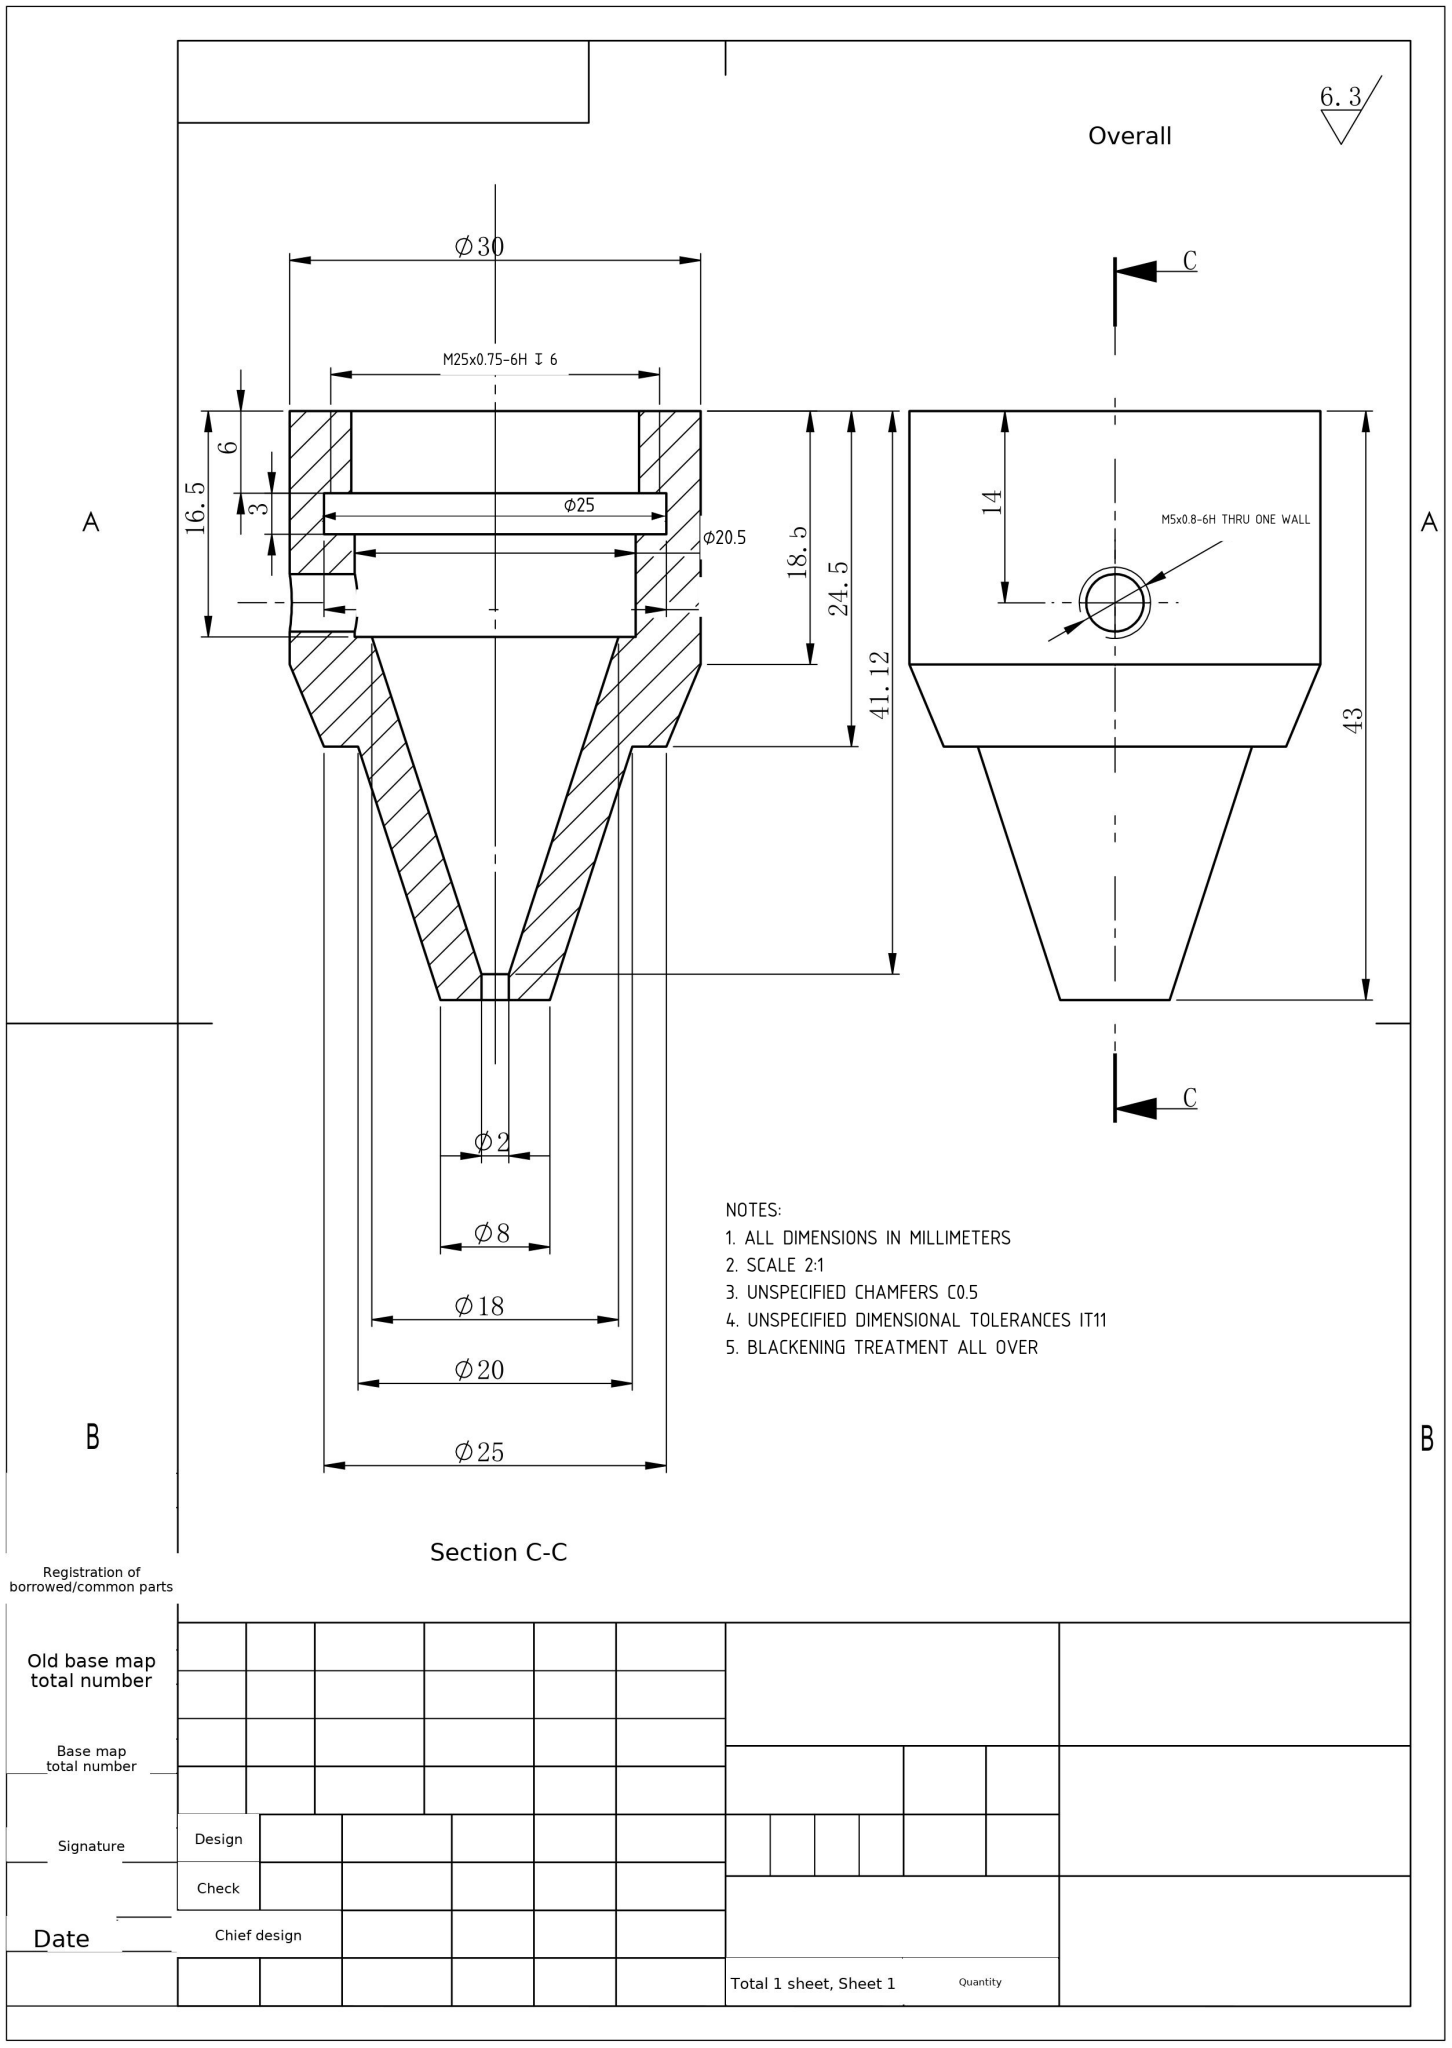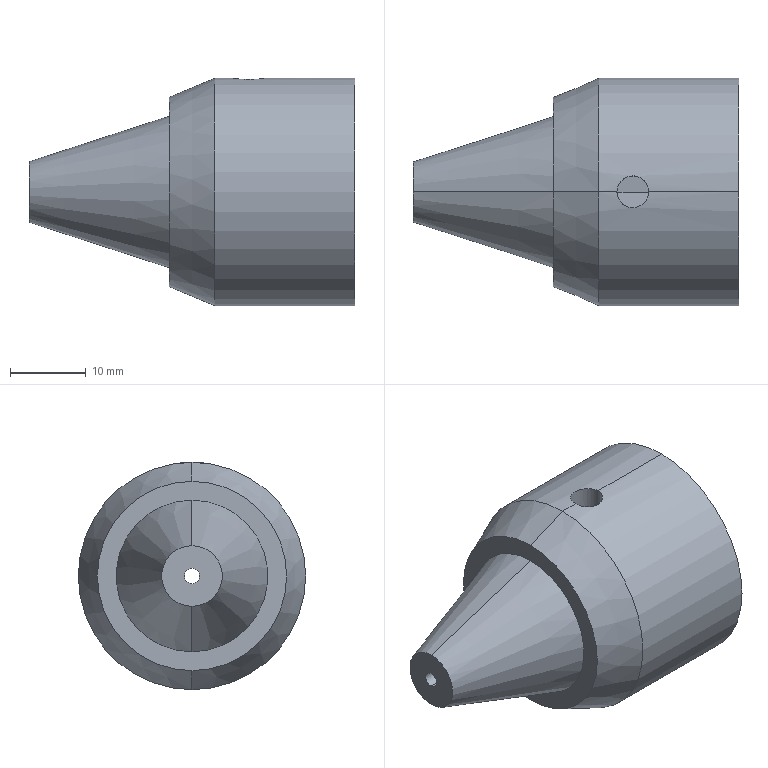Part | NX | mm | 1 solid | 24 faces | box 43 x 30 x 30 mm | volume 11233 mm3 | cylinder 12 | cone 6 | plane 6 | commonest cylinder face diameters 4.2 x2 21 x2 30 x2 2 x2 20.5 x2 25 x2
STEP:
#1=COLOUR_RGB('',0.5294,0.549,0.549);
#2=FILL_AREA_STYLE_COLOUR('',#1);
#3=FILL_AREA_STYLE('',(#2));
#4=SURFACE_STYLE_FILL_AREA(#3);
#5=SURFACE_SIDE_STYLE('',(#4));
#6=SURFACE_STYLE_USAGE(.BOTH.,#5);
#7=PRESENTATION_STYLE_ASSIGNMENT((#6));
#8=CARTESIAN_POINT('',(-9.641,-0.,10.25));
#9=VERTEX_POINT('',#8);
#10=CARTESIAN_POINT('',(-5.441,0.,10.25));
#11=VERTEX_POINT('',#10);
#12=CARTESIAN_POINT('',(-9.641,-0.,10.25));
#13=CARTESIAN_POINT('',(-9.641,-0.2744,10.25));
#14=CARTESIAN_POINT('',(-9.585,-0.5514,10.238));
#15=CARTESIAN_POINT('',(-9.428,-0.9307,10.208));
#16=CARTESIAN_POINT('',(-9.363,-1.053,10.196));
#17=CARTESIAN_POINT('',(-9.21,-1.282,10.17));
#18=CARTESIAN_POINT('',(-9.123,-1.387,10.156));
#19=CARTESIAN_POINT('',(-8.93,-1.581,10.128));
#20=CARTESIAN_POINT('',(-8.822,-1.669,10.113));
#21=CARTESIAN_POINT('',(-8.595,-1.821,10.087));
#22=CARTESIAN_POINT('',(-8.474,-1.886,10.075));
#23=CARTESIAN_POINT('',(-8.092,-2.045,10.045));
#24=CARTESIAN_POINT('',(-7.819,-2.1,10.033));
#25=CARTESIAN_POINT('',(-7.403,-2.1,10.033));
#26=CARTESIAN_POINT('',(-7.267,-2.087,10.035));
#27=CARTESIAN_POINT('',(-6.997,-2.033,10.046));
#28=CARTESIAN_POINT('',(-6.863,-1.993,10.055));
#29=CARTESIAN_POINT('',(-6.61,-1.887,10.075));
#30=CARTESIAN_POINT('',(-6.489,-1.823,10.087));
#31=CARTESIAN_POINT('',(-6.261,-1.67,10.113));
#32=CARTESIAN_POINT('',(-6.153,-1.582,10.128));
#33=CARTESIAN_POINT('',(-5.864,-1.293,10.17));
#34=CARTESIAN_POINT('',(-5.707,-1.059,10.198));
#35=CARTESIAN_POINT('',(-5.549,-0.6807,10.228));
#36=CARTESIAN_POINT('',(-5.509,-0.5474,10.236));
#37=CARTESIAN_POINT('',(-5.454,-0.2764,10.247));
#38=CARTESIAN_POINT('',(-5.441,-0.1391,10.25));
#39=CARTESIAN_POINT('',(-5.441,0.,10.25));
#40=B_SPLINE_CURVE_WITH_KNOTS('',3,(#12,#13,#14,#15,#16,#17,#18,#19,#20,#21,#22,#23,#24,#25,#26,#27,#28,#29,#30,#31,#32,#33,#34,#35,#36,#37,#38,#39),.UNSPECIFIED.,.F.,.F.,(4,2,2,2,2,2,2,2,2,2,2,2,2,4),(0.006583,0.007406,0.007817,0.008228,0.00864,0.009051,0.009874,0.01029,0.0107,0.01111,0.01152,0.01234,0.01275,0.01316),.UNSPECIFIED.);
#41=EDGE_CURVE('',#9,#11,#40,.T.);
#42=ORIENTED_EDGE('',*,*,#41,.F.);
#43=CARTESIAN_POINT('',(-9.641,0.,15.));
#44=VERTEX_POINT('',#43);
#45=CARTESIAN_POINT('',(-9.641,0.,15.));
#46=DIRECTION('',(0.,0.,1.));
#47=VECTOR('',#46,1000.);
#48=LINE('',#45,#47);
#49=EDGE_CURVE('',#9,#44,#48,.T.);
#50=ORIENTED_EDGE('',*,*,#49,.T.);
#51=CARTESIAN_POINT('',(-5.441,0.,15.));
#52=VERTEX_POINT('',#51);
#53=CARTESIAN_POINT('',(-5.441,0.,15.));
#54=CARTESIAN_POINT('',(-5.441,-0.1389,15.));
#55=CARTESIAN_POINT('',(-5.454,-0.2755,14.998));
#56=CARTESIAN_POINT('',(-5.508,-0.5442,14.991));
#57=CARTESIAN_POINT('',(-5.548,-0.6776,14.985));
#58=CARTESIAN_POINT('',(-5.654,-0.9319,14.972));
#59=CARTESIAN_POINT('',(-5.718,-1.052,14.963));
#60=CARTESIAN_POINT('',(-5.871,-1.281,14.946));
#61=CARTESIAN_POINT('',(-5.959,-1.389,14.936));
#62=CARTESIAN_POINT('',(-6.25,-1.679,14.907));
#63=CARTESIAN_POINT('',(-6.484,-1.835,14.888));
#64=CARTESIAN_POINT('',(-6.989,-2.045,14.86));
#65=CARTESIAN_POINT('',(-7.266,-2.1,14.852));
#66=CARTESIAN_POINT('',(-7.677,-2.1,14.852));
#67=CARTESIAN_POINT('',(-7.816,-2.086,14.854));
#68=CARTESIAN_POINT('',(-8.086,-2.033,14.862));
#69=CARTESIAN_POINT('',(-8.217,-1.993,14.867));
#70=CARTESIAN_POINT('',(-8.471,-1.888,14.881));
#71=CARTESIAN_POINT('',(-8.594,-1.822,14.889));
#72=CARTESIAN_POINT('',(-8.821,-1.67,14.907));
#73=CARTESIAN_POINT('',(-8.928,-1.583,14.917));
#74=CARTESIAN_POINT('',(-9.124,-1.387,14.936));
#75=CARTESIAN_POINT('',(-9.21,-1.281,14.946));
#76=CARTESIAN_POINT('',(-9.362,-1.054,14.963));
#77=CARTESIAN_POINT('',(-9.428,-0.9311,14.972));
#78=CARTESIAN_POINT('',(-9.533,-0.6769,14.985));
#79=CARTESIAN_POINT('',(-9.573,-0.5459,14.991));
#80=CARTESIAN_POINT('',(-9.627,-0.2765,14.998));
#81=CARTESIAN_POINT('',(-9.641,-0.1371,15.));
#82=CARTESIAN_POINT('',(-9.641,0.,15.));
#83=B_SPLINE_CURVE_WITH_KNOTS('',3,(#53,#54,#55,#56,#57,#58,#59,#60,#61,#62,#63,#64,#65,#66,#67,#68,#69,#70,#71,#72,#73,#74,#75,#76,#77,#78,#79,#80,#81,#82),.UNSPECIFIED.,.F.,.F.,(4,2,2,2,2,2,2,2,2,2,2,2,2,2,4),(0.,0.0004109,0.0008217,0.001233,0.001643,0.002465,0.003287,0.003698,0.004109,0.004519,0.00493,0.005341,0.005752,0.006163,0.006574),.UNSPECIFIED.);
#84=EDGE_CURVE('',#52,#44,#83,.T.);
#85=ORIENTED_EDGE('',*,*,#84,.F.);
#86=CARTESIAN_POINT('',(-5.441,0.,15.));
#87=DIRECTION('',(0.,0.,1.));
#88=VECTOR('',#87,1000.);
#89=LINE('',#86,#88);
#90=EDGE_CURVE('',#11,#52,#89,.T.);
#91=ORIENTED_EDGE('',*,*,#90,.F.);
#92=EDGE_LOOP('',(#42,#50,#85,#91));
#93=FACE_OUTER_BOUND('',#92,.T.);
#94=CARTESIAN_POINT('',(-7.541,0.,15.));
#95=DIRECTION('',(0.,0.,1.));
#96=DIRECTION('',(1.,0.,0.));
#97=AXIS2_PLACEMENT_3D('',#94,#95,#96);
#98=CYLINDRICAL_SURFACE('',#97,2.1);
#99=ADVANCED_FACE('',(#93),#98,.F.);
#100=CARTESIAN_POINT('',(0.4592,0.,10.5));
#101=VERTEX_POINT('',#100);
#102=CARTESIAN_POINT('',(0.4592,0.,-10.5));
#103=VERTEX_POINT('',#102);
#104=CARTESIAN_POINT('',(0.4592,0.,0.));
#105=DIRECTION('',(1.,0.,0.));
#106=DIRECTION('',(0.,0.,-1.));
#107=AXIS2_PLACEMENT_3D('',#104,#105,#106);
#108=CIRCLE('',#107,10.5);
#109=EDGE_CURVE('',#101,#103,#108,.T.);
#110=ORIENTED_EDGE('',*,*,#109,.F.);
#111=CARTESIAN_POINT('',(6.459,0.,10.5));
#112=VERTEX_POINT('',#111);
#113=CARTESIAN_POINT('',(6.459,0.,10.5));
#114=DIRECTION('',(1.,0.,0.));
#115=VECTOR('',#114,1000.);
#116=LINE('',#113,#115);
#117=EDGE_CURVE('',#101,#112,#116,.T.);
#118=ORIENTED_EDGE('',*,*,#117,.T.);
#119=CARTESIAN_POINT('',(6.459,0.,-10.5));
#120=VERTEX_POINT('',#119);
#121=CARTESIAN_POINT('',(6.459,0.,0.));
#122=DIRECTION('',(1.,0.,0.));
#123=DIRECTION('',(0.,0.,-1.));
#124=AXIS2_PLACEMENT_3D('',#121,#122,#123);
#125=CIRCLE('',#124,10.5);
#126=EDGE_CURVE('',#112,#120,#125,.T.);
#127=ORIENTED_EDGE('',*,*,#126,.T.);
#128=CARTESIAN_POINT('',(6.459,0.,-10.5));
#129=DIRECTION('',(1.,0.,0.));
#130=VECTOR('',#129,1000.);
#131=LINE('',#128,#130);
#132=EDGE_CURVE('',#103,#120,#131,.T.);
#133=ORIENTED_EDGE('',*,*,#132,.F.);
#134=EDGE_LOOP('',(#110,#118,#127,#133));
#135=FACE_OUTER_BOUND('',#134,.T.);
#136=CARTESIAN_POINT('',(6.459,0.,0.));
#137=DIRECTION('',(1.,0.,0.));
#138=DIRECTION('',(0.,0.,-1.));
#139=AXIS2_PLACEMENT_3D('',#136,#137,#138);
#140=CYLINDRICAL_SURFACE('',#139,10.5);
#141=ADVANCED_FACE('',(#135),#140,.F.);
#142=CARTESIAN_POINT('',(6.459,0.,15.));
#143=VERTEX_POINT('',#142);
#144=CARTESIAN_POINT('',(6.459,0.,-15.));
#145=VERTEX_POINT('',#144);
#146=CARTESIAN_POINT('',(6.459,0.,0.));
#147=DIRECTION('',(-1.,0.,0.));
#148=DIRECTION('',(0.,0.,1.));
#149=AXIS2_PLACEMENT_3D('',#146,#147,#148);
#150=CIRCLE('',#149,15.);
#151=EDGE_CURVE('',#143,#145,#150,.T.);
#152=ORIENTED_EDGE('',*,*,#151,.T.);
#153=CARTESIAN_POINT('',(-12.041,0.,-15.));
#154=VERTEX_POINT('',#153);
#155=CARTESIAN_POINT('',(-39.391,0.,-15.));
#156=DIRECTION('',(-1.,0.,0.));
#157=VECTOR('',#156,1000.);
#158=LINE('',#155,#157);
#159=EDGE_CURVE('',#145,#154,#158,.T.);
#160=ORIENTED_EDGE('',*,*,#159,.T.);
#161=CARTESIAN_POINT('',(-12.041,0.,15.));
#162=VERTEX_POINT('',#161);
#163=CARTESIAN_POINT('',(-12.041,0.,0.));
#164=DIRECTION('',(-1.,0.,0.));
#165=DIRECTION('',(0.,0.,1.));
#166=AXIS2_PLACEMENT_3D('',#163,#164,#165);
#167=CIRCLE('',#166,15.);
#168=EDGE_CURVE('',#162,#154,#167,.T.);
#169=ORIENTED_EDGE('',*,*,#168,.F.);
#170=CARTESIAN_POINT('',(-39.391,0.,15.));
#171=DIRECTION('',(-1.,0.,0.));
#172=VECTOR('',#171,1000.);
#173=LINE('',#170,#172);
#174=EDGE_CURVE('',#44,#162,#173,.T.);
#175=ORIENTED_EDGE('',*,*,#174,.F.);
#176=CARTESIAN_POINT('',(-9.641,0.,15.));
#177=CARTESIAN_POINT('',(-9.641,0.2742,15.));
#178=CARTESIAN_POINT('',(-9.586,0.5508,14.992));
#179=CARTESIAN_POINT('',(-9.429,0.9299,14.972));
#180=CARTESIAN_POINT('',(-9.363,1.052,14.963));
#181=CARTESIAN_POINT('',(-9.21,1.281,14.946));
#182=CARTESIAN_POINT('',(-9.123,1.387,14.936));
#183=CARTESIAN_POINT('',(-8.93,1.581,14.917));
#184=CARTESIAN_POINT('',(-8.822,1.669,14.907));
#185=CARTESIAN_POINT('',(-8.594,1.822,14.889));
#186=CARTESIAN_POINT('',(-8.474,1.886,14.881));
#187=CARTESIAN_POINT('',(-8.219,1.992,14.867));
#188=CARTESIAN_POINT('',(-8.086,2.033,14.862));
#189=CARTESIAN_POINT('',(-7.818,2.086,14.854));
#190=CARTESIAN_POINT('',(-7.681,2.1,14.852));
#191=CARTESIAN_POINT('',(-7.403,2.1,14.852));
#192=CARTESIAN_POINT('',(-7.267,2.087,14.854));
#193=CARTESIAN_POINT('',(-6.998,2.033,14.862));
#194=CARTESIAN_POINT('',(-6.865,1.993,14.867));
#195=CARTESIAN_POINT('',(-6.61,1.888,14.881));
#196=CARTESIAN_POINT('',(-6.49,1.823,14.889));
#197=CARTESIAN_POINT('',(-6.262,1.671,14.907));
#198=CARTESIAN_POINT('',(-6.154,1.583,14.917));
#199=CARTESIAN_POINT('',(-5.863,1.293,14.945));
#200=CARTESIAN_POINT('',(-5.707,1.059,14.965));
#201=CARTESIAN_POINT('',(-5.497,0.5538,14.992));
#202=CARTESIAN_POINT('',(-5.441,0.2778,15.));
#203=CARTESIAN_POINT('',(-5.441,0.,15.));
#204=B_SPLINE_CURVE_WITH_KNOTS('',3,(#176,#177,#178,#179,#180,#181,#182,#183,#184,#185,#186,#187,#188,#189,#190,#191,#192,#193,#194,#195,#196,#197,#198,#199,#200,#201,#202,#203),.UNSPECIFIED.,.F.,.F.,(4,2,2,2,2,2,2,2,2,2,2,2,2,4),(0.006574,0.007395,0.007806,0.008217,0.008627,0.009038,0.009449,0.00986,0.01027,0.01068,0.01109,0.0115,0.01232,0.01315),.UNSPECIFIED.);
#205=EDGE_CURVE('',#44,#52,#204,.T.);
#206=ORIENTED_EDGE('',*,*,#205,.T.);
#207=CARTESIAN_POINT('',(-39.391,0.,15.));
#208=DIRECTION('',(-1.,0.,0.));
#209=VECTOR('',#208,1000.);
#210=LINE('',#207,#209);
#211=EDGE_CURVE('',#143,#52,#210,.T.);
#212=ORIENTED_EDGE('',*,*,#211,.F.);
#213=EDGE_LOOP('',(#152,#160,#169,#175,#206,#212));
#214=FACE_OUTER_BOUND('',#213,.T.);
#215=CARTESIAN_POINT('',(-39.391,0.,0.));
#216=DIRECTION('',(-1.,0.,0.));
#217=DIRECTION('',(0.,0.,1.));
#218=AXIS2_PLACEMENT_3D('',#215,#216,#217);
#219=CYLINDRICAL_SURFACE('',#218,15.);
#220=ADVANCED_FACE('',(#214),#219,.T.);
#221=CARTESIAN_POINT('',(-18.041,0.,12.5));
#222=VERTEX_POINT('',#221);
#223=CARTESIAN_POINT('',(-18.041,0.,-12.5));
#224=VERTEX_POINT('',#223);
#225=CARTESIAN_POINT('',(-18.041,0.,0.));
#226=DIRECTION('',(-1.,0.,0.));
#227=DIRECTION('',(0.,0.,1.));
#228=AXIS2_PLACEMENT_3D('',#225,#226,#227);
#229=CIRCLE('',#228,12.5);
#230=EDGE_CURVE('',#222,#224,#229,.T.);
#231=ORIENTED_EDGE('',*,*,#230,.F.);
#232=CARTESIAN_POINT('',(-12.041,0.,15.));
#233=DIRECTION('',(0.9231,0.,0.3846));
#234=VECTOR('',#233,1000.);
#235=LINE('',#232,#234);
#236=EDGE_CURVE('',#222,#162,#235,.T.);
#237=ORIENTED_EDGE('',*,*,#236,.T.);
#238=ORIENTED_EDGE('',*,*,#168,.T.);
#239=CARTESIAN_POINT('',(-12.041,0.,-15.));
#240=DIRECTION('',(0.9231,0.,-0.3846));
#241=VECTOR('',#240,1000.);
#242=LINE('',#239,#241);
#243=EDGE_CURVE('',#224,#154,#242,.T.);
#244=ORIENTED_EDGE('',*,*,#243,.F.);
#245=EDGE_LOOP('',(#231,#237,#238,#244));
#246=FACE_OUTER_BOUND('',#245,.T.);
#247=CARTESIAN_POINT('',(-12.041,0.,0.));
#248=DIRECTION('',(1.,0.,0.));
#249=DIRECTION('',(0.,0.,-1.));
#250=AXIS2_PLACEMENT_3D('',#247,#248,#249);
#251=CONICAL_SURFACE('',#250,15.,0.3948);
#252=ADVANCED_FACE('',(#246),#251,.T.);
#253=CARTESIAN_POINT('',(-36.541,0.,4.));
#254=VERTEX_POINT('',#253);
#255=CARTESIAN_POINT('',(-36.541,0.,-4.));
#256=VERTEX_POINT('',#255);
#257=CARTESIAN_POINT('',(-36.541,0.,0.));
#258=DIRECTION('',(-1.,0.,0.));
#259=DIRECTION('',(0.,0.,1.));
#260=AXIS2_PLACEMENT_3D('',#257,#258,#259);
#261=CIRCLE('',#260,4.);
#262=EDGE_CURVE('',#254,#256,#261,.T.);
#263=ORIENTED_EDGE('',*,*,#262,.F.);
#264=CARTESIAN_POINT('',(-18.041,0.,10.011));
#265=VERTEX_POINT('',#264);
#266=CARTESIAN_POINT('',(-18.041,0.,10.011));
#267=DIRECTION('',(0.9511,0.,0.309));
#268=VECTOR('',#267,1000.);
#269=LINE('',#266,#268);
#270=EDGE_CURVE('',#254,#265,#269,.T.);
#271=ORIENTED_EDGE('',*,*,#270,.T.);
#272=CARTESIAN_POINT('',(-18.041,0.,-10.011));
#273=VERTEX_POINT('',#272);
#274=CARTESIAN_POINT('',(-18.041,0.,0.));
#275=DIRECTION('',(-1.,0.,0.));
#276=DIRECTION('',(0.,0.,1.));
#277=AXIS2_PLACEMENT_3D('',#274,#275,#276);
#278=CIRCLE('',#277,10.011);
#279=EDGE_CURVE('',#265,#273,#278,.T.);
#280=ORIENTED_EDGE('',*,*,#279,.T.);
#281=CARTESIAN_POINT('',(-18.041,0.,-10.011));
#282=DIRECTION('',(0.9511,0.,-0.309));
#283=VECTOR('',#282,1000.);
#284=LINE('',#281,#283);
#285=EDGE_CURVE('',#256,#273,#284,.T.);
#286=ORIENTED_EDGE('',*,*,#285,.F.);
#287=EDGE_LOOP('',(#263,#271,#280,#286));
#288=FACE_OUTER_BOUND('',#287,.T.);
#289=CARTESIAN_POINT('',(-18.041,0.,0.));
#290=DIRECTION('',(1.,0.,0.));
#291=DIRECTION('',(0.,0.,-1.));
#292=AXIS2_PLACEMENT_3D('',#289,#290,#291);
#293=CONICAL_SURFACE('',#292,10.011,0.3142);
#294=ADVANCED_FACE('',(#288),#293,.T.);
#295=CARTESIAN_POINT('',(-34.662,0.,-1.));
#296=VERTEX_POINT('',#295);
#297=CARTESIAN_POINT('',(-34.662,0.,1.));
#298=VERTEX_POINT('',#297);
#299=CARTESIAN_POINT('',(-34.662,0.,0.));
#300=DIRECTION('',(-1.,0.,0.));
#301=DIRECTION('',(0.,0.,1.));
#302=AXIS2_PLACEMENT_3D('',#299,#300,#301);
#303=CIRCLE('',#302,1.);
#304=EDGE_CURVE('',#296,#298,#303,.T.);
#305=ORIENTED_EDGE('',*,*,#304,.F.);
#306=CARTESIAN_POINT('',(-36.541,0.,-1.));
#307=VERTEX_POINT('',#306);
#308=CARTESIAN_POINT('',(-39.391,0.,-1.));
#309=DIRECTION('',(-1.,0.,0.));
#310=VECTOR('',#309,1000.);
#311=LINE('',#308,#310);
#312=EDGE_CURVE('',#296,#307,#311,.T.);
#313=ORIENTED_EDGE('',*,*,#312,.T.);
#314=CARTESIAN_POINT('',(-36.541,0.,1.));
#315=VERTEX_POINT('',#314);
#316=CARTESIAN_POINT('',(-36.541,0.,0.));
#317=DIRECTION('',(-1.,0.,0.));
#318=DIRECTION('',(0.,0.,1.));
#319=AXIS2_PLACEMENT_3D('',#316,#317,#318);
#320=CIRCLE('',#319,1.);
#321=EDGE_CURVE('',#307,#315,#320,.T.);
#322=ORIENTED_EDGE('',*,*,#321,.T.);
#323=CARTESIAN_POINT('',(-39.391,0.,1.));
#324=DIRECTION('',(-1.,0.,0.));
#325=VECTOR('',#324,1000.);
#326=LINE('',#323,#325);
#327=EDGE_CURVE('',#298,#315,#326,.T.);
#328=ORIENTED_EDGE('',*,*,#327,.F.);
#329=EDGE_LOOP('',(#305,#313,#322,#328));
#330=FACE_OUTER_BOUND('',#329,.T.);
#331=CARTESIAN_POINT('',(-39.391,0.,0.));
#332=DIRECTION('',(-1.,0.,0.));
#333=DIRECTION('',(0.,0.,1.));
#334=AXIS2_PLACEMENT_3D('',#331,#332,#333);
#335=CYLINDRICAL_SURFACE('',#334,1.);
#336=ADVANCED_FACE('',(#330),#335,.F.);
#337=ORIENTED_EDGE('',*,*,#304,.T.);
#338=CARTESIAN_POINT('',(-10.041,0.,9.));
#339=VERTEX_POINT('',#338);
#340=CARTESIAN_POINT('',(-34.662,0.,1.));
#341=DIRECTION('',(0.9511,0.,0.309));
#342=VECTOR('',#341,1000.);
#343=LINE('',#340,#342);
#344=EDGE_CURVE('',#298,#339,#343,.T.);
#345=ORIENTED_EDGE('',*,*,#344,.T.);
#346=CARTESIAN_POINT('',(-10.041,0.,-9.));
#347=VERTEX_POINT('',#346);
#348=CARTESIAN_POINT('',(-10.041,0.,0.));
#349=DIRECTION('',(-1.,0.,0.));
#350=DIRECTION('',(0.,0.,1.));
#351=AXIS2_PLACEMENT_3D('',#348,#349,#350);
#352=CIRCLE('',#351,9.);
#353=EDGE_CURVE('',#347,#339,#352,.T.);
#354=ORIENTED_EDGE('',*,*,#353,.F.);
#355=CARTESIAN_POINT('',(-34.662,0.,-1.));
#356=DIRECTION('',(0.9511,0.,-0.309));
#357=VECTOR('',#356,1000.);
#358=LINE('',#355,#357);
#359=EDGE_CURVE('',#296,#347,#358,.T.);
#360=ORIENTED_EDGE('',*,*,#359,.F.);
#361=EDGE_LOOP('',(#337,#345,#354,#360));
#362=FACE_OUTER_BOUND('',#361,.T.);
#363=CARTESIAN_POINT('',(-34.662,0.,0.));
#364=DIRECTION('',(1.,0.,0.));
#365=DIRECTION('',(0.,0.,-1.));
#366=AXIS2_PLACEMENT_3D('',#363,#364,#365);
#367=CONICAL_SURFACE('',#366,1.,0.3142);
#368=ADVANCED_FACE('',(#362),#367,.F.);
#369=CARTESIAN_POINT('',(-2.541,0.,-10.25));
#370=VERTEX_POINT('',#369);
#371=CARTESIAN_POINT('',(-2.541,0.,10.25));
#372=VERTEX_POINT('',#371);
#373=CARTESIAN_POINT('',(-2.541,0.,0.));
#374=DIRECTION('',(-1.,0.,0.));
#375=DIRECTION('',(0.,0.,1.));
#376=AXIS2_PLACEMENT_3D('',#373,#374,#375);
#377=CIRCLE('',#376,10.25);
#378=EDGE_CURVE('',#370,#372,#377,.T.);
#379=ORIENTED_EDGE('',*,*,#378,.F.);
#380=CARTESIAN_POINT('',(-10.041,0.,-10.25));
#381=VERTEX_POINT('',#380);
#382=CARTESIAN_POINT('',(-39.391,0.,-10.25));
#383=DIRECTION('',(-1.,0.,0.));
#384=VECTOR('',#383,1000.);
#385=LINE('',#382,#384);
#386=EDGE_CURVE('',#370,#381,#385,.T.);
#387=ORIENTED_EDGE('',*,*,#386,.T.);
#388=CARTESIAN_POINT('',(-10.041,0.,10.25));
#389=VERTEX_POINT('',#388);
#390=CARTESIAN_POINT('',(-10.041,0.,0.));
#391=DIRECTION('',(-1.,0.,0.));
#392=DIRECTION('',(0.,0.,1.));
#393=AXIS2_PLACEMENT_3D('',#390,#391,#392);
#394=CIRCLE('',#393,10.25);
#395=EDGE_CURVE('',#381,#389,#394,.T.);
#396=ORIENTED_EDGE('',*,*,#395,.T.);
#397=CARTESIAN_POINT('',(-39.391,0.,10.25));
#398=DIRECTION('',(-1.,0.,0.));
#399=VECTOR('',#398,1000.);
#400=LINE('',#397,#399);
#401=EDGE_CURVE('',#9,#389,#400,.T.);
#402=ORIENTED_EDGE('',*,*,#401,.F.);
#403=ORIENTED_EDGE('',*,*,#41,.T.);
#404=CARTESIAN_POINT('',(-39.391,0.,10.25));
#405=DIRECTION('',(-1.,0.,0.));
#406=VECTOR('',#405,1000.);
#407=LINE('',#404,#406);
#408=EDGE_CURVE('',#372,#11,#407,.T.);
#409=ORIENTED_EDGE('',*,*,#408,.F.);
#410=EDGE_LOOP('',(#379,#387,#396,#402,#403,#409));
#411=FACE_OUTER_BOUND('',#410,.T.);
#412=CARTESIAN_POINT('',(-39.391,0.,0.));
#413=DIRECTION('',(-1.,0.,0.));
#414=DIRECTION('',(0.,0.,1.));
#415=AXIS2_PLACEMENT_3D('',#412,#413,#414);
#416=CYLINDRICAL_SURFACE('',#415,10.25);
#417=ADVANCED_FACE('',(#411),#416,.F.);
#418=CARTESIAN_POINT('',(0.4592,0.,-12.5));
#419=VERTEX_POINT('',#418);
#420=CARTESIAN_POINT('',(0.4592,0.,12.5));
#421=VERTEX_POINT('',#420);
#422=CARTESIAN_POINT('',(0.4592,0.,0.));
#423=DIRECTION('',(-1.,0.,0.));
#424=DIRECTION('',(0.,0.,1.));
#425=AXIS2_PLACEMENT_3D('',#422,#423,#424);
#426=CIRCLE('',#425,12.5);
#427=EDGE_CURVE('',#419,#421,#426,.T.);
#428=ORIENTED_EDGE('',*,*,#427,.F.);
#429=CARTESIAN_POINT('',(-2.541,0.,-12.5));
#430=VERTEX_POINT('',#429);
#431=CARTESIAN_POINT('',(-39.391,0.,-12.5));
#432=DIRECTION('',(-1.,0.,0.));
#433=VECTOR('',#432,1000.);
#434=LINE('',#431,#433);
#435=EDGE_CURVE('',#419,#430,#434,.T.);
#436=ORIENTED_EDGE('',*,*,#435,.T.);
#437=CARTESIAN_POINT('',(-2.541,0.,12.5));
#438=VERTEX_POINT('',#437);
#439=CARTESIAN_POINT('',(-2.541,0.,0.));
#440=DIRECTION('',(-1.,0.,0.));
#441=DIRECTION('',(0.,0.,1.));
#442=AXIS2_PLACEMENT_3D('',#439,#440,#441);
#443=CIRCLE('',#442,12.5);
#444=EDGE_CURVE('',#430,#438,#443,.T.);
#445=ORIENTED_EDGE('',*,*,#444,.T.);
#446=CARTESIAN_POINT('',(-39.391,0.,12.5));
#447=DIRECTION('',(-1.,0.,0.));
#448=VECTOR('',#447,1000.);
#449=LINE('',#446,#448);
#450=EDGE_CURVE('',#421,#438,#449,.T.);
#451=ORIENTED_EDGE('',*,*,#450,.F.);
#452=EDGE_LOOP('',(#428,#436,#445,#451));
#453=FACE_OUTER_BOUND('',#452,.T.);
#454=CARTESIAN_POINT('',(-39.391,0.,0.));
#455=DIRECTION('',(-1.,0.,0.));
#456=DIRECTION('',(0.,0.,1.));
#457=AXIS2_PLACEMENT_3D('',#454,#455,#456);
#458=CYLINDRICAL_SURFACE('',#457,12.5);
#459=ADVANCED_FACE('',(#453),#458,.F.);
#460=CARTESIAN_POINT('',(6.459,0.,0.));
#461=DIRECTION('',(1.,0.,0.));
#462=DIRECTION('',(0.,0.,-1.));
#463=AXIS2_PLACEMENT_3D('',#460,#461,#462);
#464=CIRCLE('',#463,10.5);
#465=EDGE_CURVE('',#120,#112,#464,.T.);
#466=ORIENTED_EDGE('',*,*,#465,.F.);
#467=ORIENTED_EDGE('',*,*,#126,.F.);
#468=EDGE_LOOP('',(#466,#467));
#469=FACE_BOUND('',#468,.T.);
#470=ORIENTED_EDGE('',*,*,#151,.F.);
#471=CARTESIAN_POINT('',(6.459,0.,0.));
#472=DIRECTION('',(-1.,0.,0.));
#473=DIRECTION('',(0.,0.,1.));
#474=AXIS2_PLACEMENT_3D('',#471,#472,#473);
#475=CIRCLE('',#474,15.);
#476=EDGE_CURVE('',#145,#143,#475,.T.);
#477=ORIENTED_EDGE('',*,*,#476,.F.);
#478=EDGE_LOOP('',(#470,#477));
#479=FACE_OUTER_BOUND('',#478,.T.);
#480=CARTESIAN_POINT('',(6.459,15.,0.));
#481=DIRECTION('',(-1.,0.,0.));
#482=DIRECTION('',(0.,0.,1.));
#483=AXIS2_PLACEMENT_3D('',#480,#481,#482);
#484=PLANE('',#483);
#485=ADVANCED_FACE('',(#469,#479),#484,.F.);
#486=CARTESIAN_POINT('',(0.4592,0.,0.));
#487=DIRECTION('',(1.,0.,0.));
#488=DIRECTION('',(0.,0.,-1.));
#489=AXIS2_PLACEMENT_3D('',#486,#487,#488);
#490=CIRCLE('',#489,10.5);
#491=EDGE_CURVE('',#103,#101,#490,.T.);
#492=ORIENTED_EDGE('',*,*,#491,.T.);
#493=ORIENTED_EDGE('',*,*,#109,.T.);
#494=EDGE_LOOP('',(#492,#493));
#495=FACE_BOUND('',#494,.T.);
#496=CARTESIAN_POINT('',(0.4592,0.,0.));
#497=DIRECTION('',(-1.,0.,0.));
#498=DIRECTION('',(0.,0.,1.));
#499=AXIS2_PLACEMENT_3D('',#496,#497,#498);
#500=CIRCLE('',#499,12.5);
#501=EDGE_CURVE('',#421,#419,#500,.T.);
#502=ORIENTED_EDGE('',*,*,#501,.T.);
#503=ORIENTED_EDGE('',*,*,#427,.T.);
#504=EDGE_LOOP('',(#502,#503));
#505=FACE_OUTER_BOUND('',#504,.T.);
#506=CARTESIAN_POINT('',(0.4592,10.,0.));
#507=DIRECTION('',(1.,0.,0.));
#508=DIRECTION('',(0.,0.,-1.));
#509=AXIS2_PLACEMENT_3D('',#506,#507,#508);
#510=PLANE('',#509);
#511=ADVANCED_FACE('',(#495,#505),#510,.F.);
#512=ORIENTED_EDGE('',*,*,#435,.F.);
#513=ORIENTED_EDGE('',*,*,#501,.F.);
#514=ORIENTED_EDGE('',*,*,#450,.T.);
#515=CARTESIAN_POINT('',(-2.541,0.,0.));
#516=DIRECTION('',(-1.,0.,0.));
#517=DIRECTION('',(0.,0.,1.));
#518=AXIS2_PLACEMENT_3D('',#515,#516,#517);
#519=CIRCLE('',#518,12.5);
#520=EDGE_CURVE('',#438,#430,#519,.T.);
#521=ORIENTED_EDGE('',*,*,#520,.T.);
#522=EDGE_LOOP('',(#512,#513,#514,#521));
#523=FACE_OUTER_BOUND('',#522,.T.);
#524=CARTESIAN_POINT('',(-39.391,0.,0.));
#525=DIRECTION('',(-1.,0.,0.));
#526=DIRECTION('',(0.,0.,1.));
#527=AXIS2_PLACEMENT_3D('',#524,#525,#526);
#528=CYLINDRICAL_SURFACE('',#527,12.5);
#529=ADVANCED_FACE('',(#523),#528,.F.);
#530=ORIENTED_EDGE('',*,*,#520,.F.);
#531=ORIENTED_EDGE('',*,*,#444,.F.);
#532=EDGE_LOOP('',(#530,#531));
#533=FACE_OUTER_BOUND('',#532,.T.);
#534=CARTESIAN_POINT('',(-2.541,0.,0.));
#535=DIRECTION('',(-1.,0.,0.));
#536=DIRECTION('',(0.,0.,1.));
#537=AXIS2_PLACEMENT_3D('',#534,#535,#536);
#538=CIRCLE('',#537,10.25);
#539=EDGE_CURVE('',#372,#370,#538,.T.);
#540=ORIENTED_EDGE('',*,*,#539,.T.);
#541=ORIENTED_EDGE('',*,*,#378,.T.);
#542=EDGE_LOOP('',(#540,#541));
#543=FACE_BOUND('',#542,.T.);
#544=CARTESIAN_POINT('',(-2.541,12.5,0.));
#545=DIRECTION('',(-1.,0.,0.));
#546=DIRECTION('',(0.,0.,1.));
#547=AXIS2_PLACEMENT_3D('',#544,#545,#546);
#548=PLANE('',#547);
#549=ADVANCED_FACE('',(#533,#543),#548,.F.);
#550=ORIENTED_EDGE('',*,*,#386,.F.);
#551=ORIENTED_EDGE('',*,*,#539,.F.);
#552=ORIENTED_EDGE('',*,*,#408,.T.);
#553=CARTESIAN_POINT('',(-5.441,0.,10.25));
#554=CARTESIAN_POINT('',(-5.441,0.1391,10.25));
#555=CARTESIAN_POINT('',(-5.454,0.2759,10.247));
#556=CARTESIAN_POINT('',(-5.508,0.5448,10.236));
#557=CARTESIAN_POINT('',(-5.549,0.6784,10.228));
#558=CARTESIAN_POINT('',(-5.654,0.9326,10.208));
#559=CARTESIAN_POINT('',(-5.719,1.053,10.196));
#560=CARTESIAN_POINT('',(-5.871,1.281,10.17));
#561=CARTESIAN_POINT('',(-5.96,1.389,10.156));
#562=CARTESIAN_POINT('',(-6.249,1.678,10.114));
#563=CARTESIAN_POINT('',(-6.483,1.835,10.085));
#564=CARTESIAN_POINT('',(-6.862,1.992,10.055));
#565=CARTESIAN_POINT('',(-6.995,2.032,10.047));
#566=CARTESIAN_POINT('',(-7.266,2.087,10.035));
#567=CARTESIAN_POINT('',(-7.403,2.1,10.033));
#568=CARTESIAN_POINT('',(-7.677,2.1,10.033));
#569=CARTESIAN_POINT('',(-7.817,2.086,10.035));
#570=CARTESIAN_POINT('',(-8.087,2.032,10.047));
#571=CARTESIAN_POINT('',(-8.218,1.993,10.055));
#572=CARTESIAN_POINT('',(-8.6,1.834,10.085));
#573=CARTESIAN_POINT('',(-8.831,1.68,10.113));
#574=CARTESIAN_POINT('',(-9.123,1.387,10.156));
#575=CARTESIAN_POINT('',(-9.21,1.282,10.17));
#576=CARTESIAN_POINT('',(-9.362,1.054,10.196));
#577=CARTESIAN_POINT('',(-9.428,0.9314,10.208));
#578=CARTESIAN_POINT('',(-9.533,0.6776,10.228));
#579=CARTESIAN_POINT('',(-9.573,0.5466,10.236));
#580=CARTESIAN_POINT('',(-9.627,0.2767,10.247));
#581=CARTESIAN_POINT('',(-9.641,0.1373,10.25));
#582=CARTESIAN_POINT('',(-9.641,-0.,10.25));
#583=B_SPLINE_CURVE_WITH_KNOTS('',3,(#553,#554,#555,#556,#557,#558,#559,#560,#561,#562,#563,#564,#565,#566,#567,#568,#569,#570,#571,#572,#573,#574,#575,#576,#577,#578,#579,#580,#581,#582),.UNSPECIFIED.,.F.,.F.,(4,2,2,2,2,2,2,2,2,2,2,2,2,2,4),(0.,0.0004114,0.0008229,0.001234,0.001646,0.002469,0.00288,0.003292,0.003703,0.004114,0.004937,0.005349,0.00576,0.006172,0.006583),.UNSPECIFIED.);
#584=EDGE_CURVE('',#11,#9,#583,.T.);
#585=ORIENTED_EDGE('',*,*,#584,.T.);
#586=ORIENTED_EDGE('',*,*,#401,.T.);
#587=CARTESIAN_POINT('',(-10.041,0.,0.));
#588=DIRECTION('',(-1.,0.,0.));
#589=DIRECTION('',(0.,0.,1.));
#590=AXIS2_PLACEMENT_3D('',#587,#588,#589);
#591=CIRCLE('',#590,10.25);
#592=EDGE_CURVE('',#389,#381,#591,.T.);
#593=ORIENTED_EDGE('',*,*,#592,.T.);
#594=EDGE_LOOP('',(#550,#551,#552,#585,#586,#593));
#595=FACE_OUTER_BOUND('',#594,.T.);
#596=CARTESIAN_POINT('',(-39.391,0.,0.));
#597=DIRECTION('',(-1.,0.,0.));
#598=DIRECTION('',(0.,0.,1.));
#599=AXIS2_PLACEMENT_3D('',#596,#597,#598);
#600=CYLINDRICAL_SURFACE('',#599,10.25);
#601=ADVANCED_FACE('',(#595),#600,.F.);
#602=ORIENTED_EDGE('',*,*,#592,.F.);
#603=ORIENTED_EDGE('',*,*,#395,.F.);
#604=EDGE_LOOP('',(#602,#603));
#605=FACE_OUTER_BOUND('',#604,.T.);
#606=ORIENTED_EDGE('',*,*,#353,.T.);
#607=CARTESIAN_POINT('',(-10.041,0.,0.));
#608=DIRECTION('',(-1.,0.,0.));
#609=DIRECTION('',(0.,0.,1.));
#610=AXIS2_PLACEMENT_3D('',#607,#608,#609);
#611=CIRCLE('',#610,9.);
#612=EDGE_CURVE('',#339,#347,#611,.T.);
#613=ORIENTED_EDGE('',*,*,#612,.T.);
#614=EDGE_LOOP('',(#606,#613));
#615=FACE_BOUND('',#614,.T.);
#616=CARTESIAN_POINT('',(-10.041,10.25,0.));
#617=DIRECTION('',(-1.,0.,0.));
#618=DIRECTION('',(0.,0.,1.));
#619=AXIS2_PLACEMENT_3D('',#616,#617,#618);
#620=PLANE('',#619);
#621=ADVANCED_FACE('',(#605,#615),#620,.F.);
#622=ORIENTED_EDGE('',*,*,#344,.F.);
#623=CARTESIAN_POINT('',(-34.662,0.,0.));
#624=DIRECTION('',(-1.,0.,0.));
#625=DIRECTION('',(0.,0.,1.));
#626=AXIS2_PLACEMENT_3D('',#623,#624,#625);
#627=CIRCLE('',#626,1.);
#628=EDGE_CURVE('',#298,#296,#627,.T.);
#629=ORIENTED_EDGE('',*,*,#628,.T.);
#630=ORIENTED_EDGE('',*,*,#359,.T.);
#631=ORIENTED_EDGE('',*,*,#612,.F.);
#632=EDGE_LOOP('',(#622,#629,#630,#631));
#633=FACE_OUTER_BOUND('',#632,.T.);
#634=CARTESIAN_POINT('',(-34.662,0.,0.));
#635=DIRECTION('',(1.,0.,0.));
#636=DIRECTION('',(0.,0.,-1.));
#637=AXIS2_PLACEMENT_3D('',#634,#635,#636);
#638=CONICAL_SURFACE('',#637,1.,0.3142);
#639=ADVANCED_FACE('',(#633),#638,.F.);
#640=ORIENTED_EDGE('',*,*,#312,.F.);
#641=ORIENTED_EDGE('',*,*,#628,.F.);
#642=ORIENTED_EDGE('',*,*,#327,.T.);
#643=CARTESIAN_POINT('',(-36.541,0.,0.));
#644=DIRECTION('',(-1.,0.,0.));
#645=DIRECTION('',(0.,0.,1.));
#646=AXIS2_PLACEMENT_3D('',#643,#644,#645);
#647=CIRCLE('',#646,1.);
#648=EDGE_CURVE('',#315,#307,#647,.T.);
#649=ORIENTED_EDGE('',*,*,#648,.T.);
#650=EDGE_LOOP('',(#640,#641,#642,#649));
#651=FACE_OUTER_BOUND('',#650,.T.);
#652=CARTESIAN_POINT('',(-39.391,0.,0.));
#653=DIRECTION('',(-1.,0.,0.));
#654=DIRECTION('',(0.,0.,1.));
#655=AXIS2_PLACEMENT_3D('',#652,#653,#654);
#656=CYLINDRICAL_SURFACE('',#655,1.);
#657=ADVANCED_FACE('',(#651),#656,.F.);
#658=ORIENTED_EDGE('',*,*,#648,.F.);
#659=ORIENTED_EDGE('',*,*,#321,.F.);
#660=EDGE_LOOP('',(#658,#659));
#661=FACE_BOUND('',#660,.T.);
#662=CARTESIAN_POINT('',(-36.541,0.,0.));
#663=DIRECTION('',(-1.,0.,0.));
#664=DIRECTION('',(0.,0.,1.));
#665=AXIS2_PLACEMENT_3D('',#662,#663,#664);
#666=CIRCLE('',#665,4.);
#667=EDGE_CURVE('',#256,#254,#666,.T.);
#668=ORIENTED_EDGE('',*,*,#667,.T.);
#669=ORIENTED_EDGE('',*,*,#262,.T.);
#670=EDGE_LOOP('',(#668,#669));
#671=FACE_OUTER_BOUND('',#670,.T.);
#672=CARTESIAN_POINT('',(-36.541,1.,0.));
#673=DIRECTION('',(1.,0.,0.));
#674=DIRECTION('',(0.,0.,-1.));
#675=AXIS2_PLACEMENT_3D('',#672,#673,#674);
#676=PLANE('',#675);
#677=ADVANCED_FACE('',(#661,#671),#676,.F.);
#678=ORIENTED_EDGE('',*,*,#270,.F.);
#679=ORIENTED_EDGE('',*,*,#667,.F.);
#680=ORIENTED_EDGE('',*,*,#285,.T.);
#681=CARTESIAN_POINT('',(-18.041,0.,0.));
#682=DIRECTION('',(-1.,0.,0.));
#683=DIRECTION('',(0.,0.,1.));
#684=AXIS2_PLACEMENT_3D('',#681,#682,#683);
#685=CIRCLE('',#684,10.011);
#686=EDGE_CURVE('',#273,#265,#685,.T.);
#687=ORIENTED_EDGE('',*,*,#686,.T.);
#688=EDGE_LOOP('',(#678,#679,#680,#687));
#689=FACE_OUTER_BOUND('',#688,.T.);
#690=CARTESIAN_POINT('',(-18.041,0.,0.));
#691=DIRECTION('',(1.,0.,0.));
#692=DIRECTION('',(0.,0.,-1.));
#693=AXIS2_PLACEMENT_3D('',#690,#691,#692);
#694=CONICAL_SURFACE('',#693,10.011,0.3142);
#695=ADVANCED_FACE('',(#689),#694,.T.);
#696=ORIENTED_EDGE('',*,*,#686,.F.);
#697=ORIENTED_EDGE('',*,*,#279,.F.);
#698=EDGE_LOOP('',(#696,#697));
#699=FACE_BOUND('',#698,.T.);
#700=CARTESIAN_POINT('',(-18.041,0.,0.));
#701=DIRECTION('',(-1.,0.,0.));
#702=DIRECTION('',(0.,0.,1.));
#703=AXIS2_PLACEMENT_3D('',#700,#701,#702);
#704=CIRCLE('',#703,12.5);
#705=EDGE_CURVE('',#224,#222,#704,.T.);
#706=ORIENTED_EDGE('',*,*,#705,.T.);
#707=ORIENTED_EDGE('',*,*,#230,.T.);
#708=EDGE_LOOP('',(#706,#707));
#709=FACE_OUTER_BOUND('',#708,.T.);
#710=CARTESIAN_POINT('',(-18.041,10.011,0.));
#711=DIRECTION('',(1.,0.,0.));
#712=DIRECTION('',(0.,0.,-1.));
#713=AXIS2_PLACEMENT_3D('',#710,#711,#712);
#714=PLANE('',#713);
#715=ADVANCED_FACE('',(#699,#709),#714,.F.);
#716=ORIENTED_EDGE('',*,*,#236,.F.);
#717=ORIENTED_EDGE('',*,*,#705,.F.);
#718=ORIENTED_EDGE('',*,*,#243,.T.);
#719=CARTESIAN_POINT('',(-12.041,0.,0.));
#720=DIRECTION('',(-1.,0.,0.));
#721=DIRECTION('',(0.,0.,1.));
#722=AXIS2_PLACEMENT_3D('',#719,#720,#721);
#723=CIRCLE('',#722,15.);
#724=EDGE_CURVE('',#154,#162,#723,.T.);
#725=ORIENTED_EDGE('',*,*,#724,.T.);
#726=EDGE_LOOP('',(#716,#717,#718,#725));
#727=FACE_OUTER_BOUND('',#726,.T.);
#728=CARTESIAN_POINT('',(-12.041,0.,0.));
#729=DIRECTION('',(1.,0.,0.));
#730=DIRECTION('',(0.,0.,-1.));
#731=AXIS2_PLACEMENT_3D('',#728,#729,#730);
#732=CONICAL_SURFACE('',#731,15.,0.3948);
#733=ADVANCED_FACE('',(#727),#732,.T.);
#734=ORIENTED_EDGE('',*,*,#159,.F.);
#735=ORIENTED_EDGE('',*,*,#476,.T.);
#736=ORIENTED_EDGE('',*,*,#211,.T.);
#737=ORIENTED_EDGE('',*,*,#84,.T.);
#738=ORIENTED_EDGE('',*,*,#174,.T.);
#739=ORIENTED_EDGE('',*,*,#724,.F.);
#740=EDGE_LOOP('',(#734,#735,#736,#737,#738,#739));
#741=FACE_OUTER_BOUND('',#740,.T.);
#742=CARTESIAN_POINT('',(-39.391,0.,0.));
#743=DIRECTION('',(-1.,0.,0.));
#744=DIRECTION('',(0.,0.,1.));
#745=AXIS2_PLACEMENT_3D('',#742,#743,#744);
#746=CYLINDRICAL_SURFACE('',#745,15.);
#747=ADVANCED_FACE('',(#741),#746,.T.);
#748=ORIENTED_EDGE('',*,*,#117,.F.);
#749=ORIENTED_EDGE('',*,*,#491,.F.);
#750=ORIENTED_EDGE('',*,*,#132,.T.);
#751=ORIENTED_EDGE('',*,*,#465,.T.);
#752=EDGE_LOOP('',(#748,#749,#750,#751));
#753=FACE_OUTER_BOUND('',#752,.T.);
#754=CARTESIAN_POINT('',(6.459,0.,0.));
#755=DIRECTION('',(1.,0.,0.));
#756=DIRECTION('',(0.,0.,-1.));
#757=AXIS2_PLACEMENT_3D('',#754,#755,#756);
#758=CYLINDRICAL_SURFACE('',#757,10.5);
#759=ADVANCED_FACE('',(#753),#758,.F.);
#760=ORIENTED_EDGE('',*,*,#49,.F.);
#761=ORIENTED_EDGE('',*,*,#584,.F.);
#762=ORIENTED_EDGE('',*,*,#90,.T.);
#763=ORIENTED_EDGE('',*,*,#205,.F.);
#764=EDGE_LOOP('',(#760,#761,#762,#763));
#765=FACE_OUTER_BOUND('',#764,.T.);
#766=CARTESIAN_POINT('',(-7.541,0.,15.));
#767=DIRECTION('',(0.,0.,1.));
#768=DIRECTION('',(1.,0.,0.));
#769=AXIS2_PLACEMENT_3D('',#766,#767,#768);
#770=CYLINDRICAL_SURFACE('',#769,2.1);
#771=ADVANCED_FACE('',(#765),#770,.F.);
#772=CLOSED_SHELL('',(#99,#141,#220,#252,#294,#336,#368,#417,#459,#485,#511,#529,#549,#601,#621,#639,#657,#677,#695,#715,#733,#747,#759,#771));
#773=MANIFOLD_SOLID_BREP('',#772);
#774=STYLED_ITEM('',(#7),#773);
#775=PRESENTATION_LAYER_ASSIGNMENT('','',(#774));
#776=COLOUR_RGB('',0.5294,0.549,0.549);
#777=FILL_AREA_STYLE_COLOUR('',#776);
#778=FILL_AREA_STYLE('',(#777));
#779=SURFACE_STYLE_FILL_AREA(#778);
#780=SURFACE_SIDE_STYLE('',(#779));
#781=SURFACE_STYLE_USAGE(.BOTH.,#780);
#782=PRESENTATION_STYLE_ASSIGNMENT((#781));
#783=STYLED_ITEM('',(#782),#759);
#784=(LENGTH_UNIT()NAMED_UNIT(*)SI_UNIT(.MILLI.,.METRE.));
#785=UNCERTAINTY_MEASURE_WITH_UNIT(LENGTH_MEASURE(0.00001),#784,'','');
#786=(NAMED_UNIT(*)PLANE_ANGLE_UNIT()SI_UNIT($,.RADIAN.));
#787=(NAMED_UNIT(*)SI_UNIT($,.STERADIAN.)SOLID_ANGLE_UNIT());
#788=(GEOMETRIC_REPRESENTATION_CONTEXT(3)GLOBAL_UNCERTAINTY_ASSIGNED_CONTEXT((#785))GLOBAL_UNIT_ASSIGNED_CONTEXT((#784,#786,#787))REPRESENTATION_CONTEXT('',''));
#789=MECHANICAL_DESIGN_GEOMETRIC_PRESENTATION_REPRESENTATION('',(#783),#788);
#790=(LENGTH_UNIT()NAMED_UNIT(*)SI_UNIT(.MILLI.,.METRE.));
#791=UNCERTAINTY_MEASURE_WITH_UNIT(LENGTH_MEASURE(0.00001),#790,'','');
#792=(NAMED_UNIT(*)PLANE_ANGLE_UNIT()SI_UNIT($,.RADIAN.));
#793=(NAMED_UNIT(*)SI_UNIT($,.STERADIAN.)SOLID_ANGLE_UNIT());
#794=(GEOMETRIC_REPRESENTATION_CONTEXT(3)GLOBAL_UNCERTAINTY_ASSIGNED_CONTEXT((#791))GLOBAL_UNIT_ASSIGNED_CONTEXT((#790,#792,#793))REPRESENTATION_CONTEXT('',''));
#795=MECHANICAL_DESIGN_GEOMETRIC_PRESENTATION_REPRESENTATION('',(#774),#794);
#796=COLOUR_RGB('',0.5294,0.549,0.549);
#797=FILL_AREA_STYLE_COLOUR('',#796);
#798=FILL_AREA_STYLE('',(#797));
#799=SURFACE_STYLE_FILL_AREA(#798);
#800=SURFACE_SIDE_STYLE('',(#799));
#801=SURFACE_STYLE_USAGE(.BOTH.,#800);
#802=PRESENTATION_STYLE_ASSIGNMENT((#801));
#803=CARTESIAN_POINT('',(0.,0.,0.));
#804=DIRECTION('',(0.,0.,1.));
#805=DIRECTION('',(1.,0.,0.));
#806=AXIS2_PLACEMENT_3D('',#803,#804,#805);
#807=(LENGTH_UNIT()NAMED_UNIT(*)SI_UNIT(.MILLI.,.METRE.));
#808=UNCERTAINTY_MEASURE_WITH_UNIT(LENGTH_MEASURE(0.00001),#807,'','');
#809=(NAMED_UNIT(*)PLANE_ANGLE_UNIT()SI_UNIT($,.RADIAN.));
#810=(NAMED_UNIT(*)SI_UNIT($,.STERADIAN.)SOLID_ANGLE_UNIT());
#811=(GEOMETRIC_REPRESENTATION_CONTEXT(3)GLOBAL_UNCERTAINTY_ASSIGNED_CONTEXT((#808))GLOBAL_UNIT_ASSIGNED_CONTEXT((#807,#809,#810))REPRESENTATION_CONTEXT('',''));
#812=ADVANCED_BREP_SHAPE_REPRESENTATION('',(#773,#806),#811);
#813=STYLED_ITEM('',(#802),#812);
#814=PRESENTATION_LAYER_ASSIGNMENT('','',(#813));
#815=PRESENTATION_LAYER_ASSIGNMENT('','',(#783));
#816=COLOUR_RGB('',0.5294,0.549,0.549);
#817=FILL_AREA_STYLE_COLOUR('',#816);
#818=FILL_AREA_STYLE('',(#817));
#819=SURFACE_STYLE_FILL_AREA(#818);
#820=SURFACE_SIDE_STYLE('',(#819));
#821=SURFACE_STYLE_USAGE(.BOTH.,#820);
#822=PRESENTATION_STYLE_ASSIGNMENT((#821));
#823=STYLED_ITEM('',(#822),#141);
#824=PRESENTATION_LAYER_ASSIGNMENT('','',(#823));
#825=(LENGTH_UNIT()NAMED_UNIT(*)SI_UNIT(.MILLI.,.METRE.));
#826=UNCERTAINTY_MEASURE_WITH_UNIT(LENGTH_MEASURE(0.00001),#825,'','');
#827=(NAMED_UNIT(*)PLANE_ANGLE_UNIT()SI_UNIT($,.RADIAN.));
#828=(NAMED_UNIT(*)SI_UNIT($,.STERADIAN.)SOLID_ANGLE_UNIT());
#829=(GEOMETRIC_REPRESENTATION_CONTEXT(3)GLOBAL_UNCERTAINTY_ASSIGNED_CONTEXT((#826))GLOBAL_UNIT_ASSIGNED_CONTEXT((#825,#827,#828))REPRESENTATION_CONTEXT('',''));
#830=MECHANICAL_DESIGN_GEOMETRIC_PRESENTATION_REPRESENTATION('',(#823),#829);
#831=(LENGTH_UNIT()NAMED_UNIT(*)SI_UNIT(.MILLI.,.METRE.));
#832=UNCERTAINTY_MEASURE_WITH_UNIT(LENGTH_MEASURE(0.00001),#831,'','');
#833=(NAMED_UNIT(*)PLANE_ANGLE_UNIT()SI_UNIT($,.RADIAN.));
#834=(NAMED_UNIT(*)SI_UNIT($,.STERADIAN.)SOLID_ANGLE_UNIT());
#835=(GEOMETRIC_REPRESENTATION_CONTEXT(3)GLOBAL_UNCERTAINTY_ASSIGNED_CONTEXT((#832))GLOBAL_UNIT_ASSIGNED_CONTEXT((#831,#833,#834))REPRESENTATION_CONTEXT('',''));
#836=MECHANICAL_DESIGN_GEOMETRIC_PRESENTATION_REPRESENTATION('',(#813),#835);